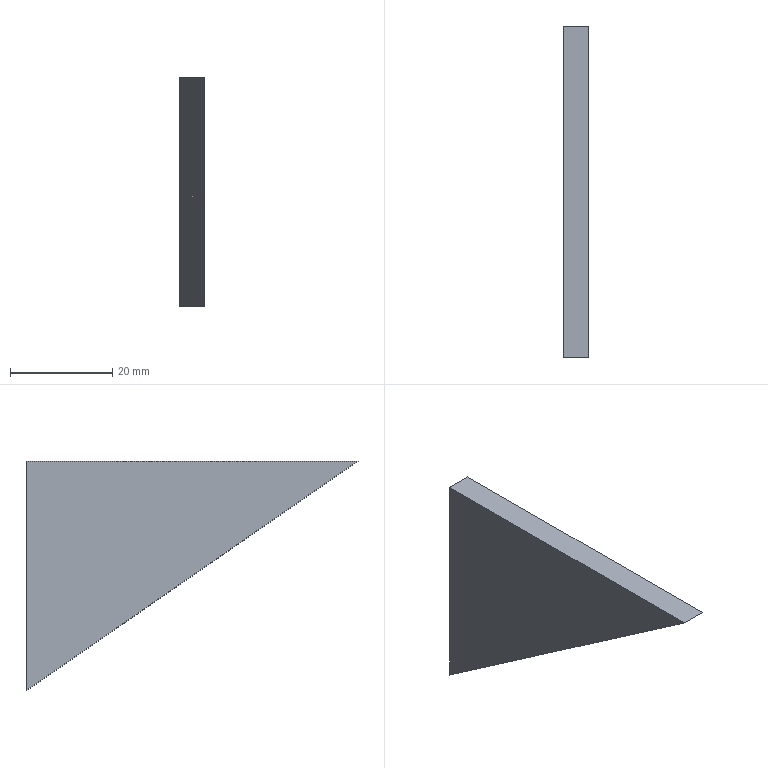Component | NX | FIXED_PLATE_13 | 1 solid | 5 faces | box 5 x 65 x 45 mm | volume 7312 mm3 | plane 5
STEP:
#1=CARTESIAN_POINT('',(0.,0.,0.));
#2=DIRECTION('',(0.,0.,1.));
#3=DIRECTION('',(1.,0.,0.));
#4=AXIS2_PLACEMENT_3D('',#1,#2,#3);
#5=CARTESIAN_POINT('',(1469.254,1356.,781.574));
#6=VERTEX_POINT('',#5);
#7=CARTESIAN_POINT('',(1469.254,1421.,736.574));
#8=VERTEX_POINT('',#7);
#9=CARTESIAN_POINT('',(1469.254,1356.,781.574));
#10=DIRECTION('',(0.,0.8222,-0.5692));
#11=VECTOR('',#10,1.);
#12=LINE('',#9,#11);
#13=CARTESIAN_POINT('',(1464.254,1356.,781.574));
#14=DIRECTION('',(0.,-0.5692,-0.8222));
#15=DIRECTION('',(0.,0.8222,-0.5692));
#16=AXIS2_PLACEMENT_3D('',#13,#14,#15);
#17=PLANE('',#16);
#18=CARTESIAN_POINT('',(0.,5.));
#19=DIRECTION('',(1.,0.));
#20=VECTOR('',#19,1.);
#21=LINE('',#18,#20);
#22=(GEOMETRIC_REPRESENTATION_CONTEXT(2)PARAMETRIC_REPRESENTATION_CONTEXT()REPRESENTATION_CONTEXT('',''));
#23=DEFINITIONAL_REPRESENTATION('',(#21),#22);
#24=PCURVE('',#17,#23);
#25=CARTESIAN_POINT('',(1469.254,0.,0.));
#26=DIRECTION('',(1.,0.,0.));
#27=DIRECTION('',(0.,0.,-1.));
#28=AXIS2_PLACEMENT_3D('',#25,#26,#27);
#29=PLANE('',#28);
#30=CARTESIAN_POINT('',(-781.574,1356.));
#31=DIRECTION('',(0.5692,0.8222));
#32=VECTOR('',#31,1.);
#33=LINE('',#30,#32);
#34=(GEOMETRIC_REPRESENTATION_CONTEXT(2)PARAMETRIC_REPRESENTATION_CONTEXT()REPRESENTATION_CONTEXT('',''));
#35=DEFINITIONAL_REPRESENTATION('',(#33),#34);
#36=PCURVE('',#29,#35);
#37=SURFACE_CURVE('',#12,(#24,#36),.PCURVE_S1.);
#38=EDGE_CURVE('',#6,#8,#37,.T.);
#39=ORIENTED_EDGE('',*,*,#38,.F.);
#40=CARTESIAN_POINT('',(1464.254,1356.,781.574));
#41=VERTEX_POINT('',#40);
#42=CARTESIAN_POINT('',(1464.254,1356.,781.574));
#43=DIRECTION('',(1.,0.,0.));
#44=VECTOR('',#43,1.);
#45=LINE('',#42,#44);
#46=CARTESIAN_POINT('',(0.,0.));
#47=DIRECTION('',(0.,1.));
#48=VECTOR('',#47,1.);
#49=LINE('',#46,#48);
#50=(GEOMETRIC_REPRESENTATION_CONTEXT(2)PARAMETRIC_REPRESENTATION_CONTEXT()REPRESENTATION_CONTEXT('',''));
#51=DEFINITIONAL_REPRESENTATION('',(#49),#50);
#52=PCURVE('',#17,#51);
#53=CARTESIAN_POINT('',(1464.254,1421.,781.574));
#54=DIRECTION('',(0.,0.,1.));
#55=DIRECTION('',(1.,0.,0.));
#56=AXIS2_PLACEMENT_3D('',#53,#54,#55);
#57=PLANE('',#56);
#58=CARTESIAN_POINT('',(0.,-65.));
#59=DIRECTION('',(1.,0.));
#60=VECTOR('',#59,1.);
#61=LINE('',#58,#60);
#62=(GEOMETRIC_REPRESENTATION_CONTEXT(2)PARAMETRIC_REPRESENTATION_CONTEXT()REPRESENTATION_CONTEXT('',''));
#63=DEFINITIONAL_REPRESENTATION('',(#61),#62);
#64=PCURVE('',#57,#63);
#65=SURFACE_CURVE('',#45,(#52,#64),.PCURVE_S1.);
#66=EDGE_CURVE('',#41,#6,#65,.T.);
#67=ORIENTED_EDGE('',*,*,#66,.F.);
#68=CARTESIAN_POINT('',(1464.254,1421.,736.574));
#69=VERTEX_POINT('',#68);
#70=CARTESIAN_POINT('',(1464.254,1356.,781.574));
#71=DIRECTION('',(0.,0.8222,-0.5692));
#72=VECTOR('',#71,1.);
#73=LINE('',#70,#72);
#74=CARTESIAN_POINT('',(0.,0.));
#75=DIRECTION('',(1.,0.));
#76=VECTOR('',#75,1.);
#77=LINE('',#74,#76);
#78=(GEOMETRIC_REPRESENTATION_CONTEXT(2)PARAMETRIC_REPRESENTATION_CONTEXT()REPRESENTATION_CONTEXT('',''));
#79=DEFINITIONAL_REPRESENTATION('',(#77),#78);
#80=PCURVE('',#17,#79);
#81=CARTESIAN_POINT('',(1464.254,0.,0.));
#82=DIRECTION('',(1.,0.,0.));
#83=DIRECTION('',(0.,0.,-1.));
#84=AXIS2_PLACEMENT_3D('',#81,#82,#83);
#85=PLANE('',#84);
#86=CARTESIAN_POINT('',(-781.574,1356.));
#87=DIRECTION('',(0.5692,0.8222));
#88=VECTOR('',#87,1.);
#89=LINE('',#86,#88);
#90=(GEOMETRIC_REPRESENTATION_CONTEXT(2)PARAMETRIC_REPRESENTATION_CONTEXT()REPRESENTATION_CONTEXT('',''));
#91=DEFINITIONAL_REPRESENTATION('',(#89),#90);
#92=PCURVE('',#85,#91);
#93=SURFACE_CURVE('',#73,(#80,#92),.PCURVE_S1.);
#94=EDGE_CURVE('',#41,#69,#93,.T.);
#95=ORIENTED_EDGE('',*,*,#94,.T.);
#96=CARTESIAN_POINT('',(1464.254,1421.,736.574));
#97=DIRECTION('',(1.,0.,0.));
#98=VECTOR('',#97,1.);
#99=LINE('',#96,#98);
#100=CARTESIAN_POINT('',(79.057,0.));
#101=DIRECTION('',(0.,1.));
#102=VECTOR('',#101,1.);
#103=LINE('',#100,#102);
#104=(GEOMETRIC_REPRESENTATION_CONTEXT(2)PARAMETRIC_REPRESENTATION_CONTEXT()REPRESENTATION_CONTEXT('',''));
#105=DEFINITIONAL_REPRESENTATION('',(#103),#104);
#106=PCURVE('',#17,#105);
#107=CARTESIAN_POINT('',(1464.254,1421.,736.574));
#108=DIRECTION('',(0.,1.,0.));
#109=DIRECTION('',(0.,0.,1.));
#110=AXIS2_PLACEMENT_3D('',#107,#108,#109);
#111=PLANE('',#110);
#112=CARTESIAN_POINT('',(0.,0.));
#113=DIRECTION('',(0.,1.));
#114=VECTOR('',#113,1.);
#115=LINE('',#112,#114);
#116=(GEOMETRIC_REPRESENTATION_CONTEXT(2)PARAMETRIC_REPRESENTATION_CONTEXT()REPRESENTATION_CONTEXT('',''));
#117=DEFINITIONAL_REPRESENTATION('',(#115),#116);
#118=PCURVE('',#111,#117);
#119=SURFACE_CURVE('',#99,(#106,#118),.PCURVE_S1.);
#120=EDGE_CURVE('',#69,#8,#119,.T.);
#121=ORIENTED_EDGE('',*,*,#120,.T.);
#122=EDGE_LOOP('',(#39,#67,#95,#121));
#123=FACE_BOUND('',#122,.T.);
#124=ADVANCED_FACE('',(#123),#17,.T.);
#125=CARTESIAN_POINT('',(1469.254,1421.,781.574));
#126=VERTEX_POINT('',#125);
#127=CARTESIAN_POINT('',(1469.254,1421.,736.574));
#128=DIRECTION('',(0.,0.,1.));
#129=VECTOR('',#128,1.);
#130=LINE('',#127,#129);
#131=CARTESIAN_POINT('',(0.,5.));
#132=DIRECTION('',(1.,0.));
#133=VECTOR('',#132,1.);
#134=LINE('',#131,#133);
#135=(GEOMETRIC_REPRESENTATION_CONTEXT(2)PARAMETRIC_REPRESENTATION_CONTEXT()REPRESENTATION_CONTEXT('',''));
#136=DEFINITIONAL_REPRESENTATION('',(#134),#135);
#137=PCURVE('',#111,#136);
#138=CARTESIAN_POINT('',(-736.574,1421.));
#139=DIRECTION('',(-1.,0.));
#140=VECTOR('',#139,1.);
#141=LINE('',#138,#140);
#142=(GEOMETRIC_REPRESENTATION_CONTEXT(2)PARAMETRIC_REPRESENTATION_CONTEXT()REPRESENTATION_CONTEXT('',''));
#143=DEFINITIONAL_REPRESENTATION('',(#141),#142);
#144=PCURVE('',#29,#143);
#145=SURFACE_CURVE('',#130,(#137,#144),.PCURVE_S1.);
#146=EDGE_CURVE('',#8,#126,#145,.T.);
#147=ORIENTED_EDGE('',*,*,#146,.F.);
#148=ORIENTED_EDGE('',*,*,#120,.F.);
#149=CARTESIAN_POINT('',(1464.254,1421.,781.574));
#150=VERTEX_POINT('',#149);
#151=CARTESIAN_POINT('',(1464.254,1421.,736.574));
#152=DIRECTION('',(0.,0.,1.));
#153=VECTOR('',#152,1.);
#154=LINE('',#151,#153);
#155=CARTESIAN_POINT('',(0.,0.));
#156=DIRECTION('',(1.,0.));
#157=VECTOR('',#156,1.);
#158=LINE('',#155,#157);
#159=(GEOMETRIC_REPRESENTATION_CONTEXT(2)PARAMETRIC_REPRESENTATION_CONTEXT()REPRESENTATION_CONTEXT('',''));
#160=DEFINITIONAL_REPRESENTATION('',(#158),#159);
#161=PCURVE('',#111,#160);
#162=CARTESIAN_POINT('',(-736.574,1421.));
#163=DIRECTION('',(-1.,0.));
#164=VECTOR('',#163,1.);
#165=LINE('',#162,#164);
#166=(GEOMETRIC_REPRESENTATION_CONTEXT(2)PARAMETRIC_REPRESENTATION_CONTEXT()REPRESENTATION_CONTEXT('',''));
#167=DEFINITIONAL_REPRESENTATION('',(#165),#166);
#168=PCURVE('',#85,#167);
#169=SURFACE_CURVE('',#154,(#161,#168),.PCURVE_S1.);
#170=EDGE_CURVE('',#69,#150,#169,.T.);
#171=ORIENTED_EDGE('',*,*,#170,.T.);
#172=CARTESIAN_POINT('',(1464.254,1421.,781.574));
#173=DIRECTION('',(1.,0.,0.));
#174=VECTOR('',#173,1.);
#175=LINE('',#172,#174);
#176=CARTESIAN_POINT('',(45.,0.));
#177=DIRECTION('',(0.,1.));
#178=VECTOR('',#177,1.);
#179=LINE('',#176,#178);
#180=(GEOMETRIC_REPRESENTATION_CONTEXT(2)PARAMETRIC_REPRESENTATION_CONTEXT()REPRESENTATION_CONTEXT('',''));
#181=DEFINITIONAL_REPRESENTATION('',(#179),#180);
#182=PCURVE('',#111,#181);
#183=CARTESIAN_POINT('',(0.,0.));
#184=DIRECTION('',(1.,0.));
#185=VECTOR('',#184,1.);
#186=LINE('',#183,#185);
#187=(GEOMETRIC_REPRESENTATION_CONTEXT(2)PARAMETRIC_REPRESENTATION_CONTEXT()REPRESENTATION_CONTEXT('',''));
#188=DEFINITIONAL_REPRESENTATION('',(#186),#187);
#189=PCURVE('',#57,#188);
#190=SURFACE_CURVE('',#175,(#182,#189),.PCURVE_S1.);
#191=EDGE_CURVE('',#150,#126,#190,.T.);
#192=ORIENTED_EDGE('',*,*,#191,.T.);
#193=EDGE_LOOP('',(#147,#148,#171,#192));
#194=FACE_BOUND('',#193,.T.);
#195=ADVANCED_FACE('',(#194),#111,.T.);
#196=CARTESIAN_POINT('',(1469.254,1421.,781.574));
#197=DIRECTION('',(0.,-1.,0.));
#198=VECTOR('',#197,1.);
#199=LINE('',#196,#198);
#200=CARTESIAN_POINT('',(5.,0.));
#201=DIRECTION('',(0.,-1.));
#202=VECTOR('',#201,1.);
#203=LINE('',#200,#202);
#204=(GEOMETRIC_REPRESENTATION_CONTEXT(2)PARAMETRIC_REPRESENTATION_CONTEXT()REPRESENTATION_CONTEXT('',''));
#205=DEFINITIONAL_REPRESENTATION('',(#203),#204);
#206=PCURVE('',#57,#205);
#207=CARTESIAN_POINT('',(-781.574,1421.));
#208=DIRECTION('',(0.,-1.));
#209=VECTOR('',#208,1.);
#210=LINE('',#207,#209);
#211=(GEOMETRIC_REPRESENTATION_CONTEXT(2)PARAMETRIC_REPRESENTATION_CONTEXT()REPRESENTATION_CONTEXT('',''));
#212=DEFINITIONAL_REPRESENTATION('',(#210),#211);
#213=PCURVE('',#29,#212);
#214=SURFACE_CURVE('',#199,(#206,#213),.PCURVE_S1.);
#215=EDGE_CURVE('',#126,#6,#214,.T.);
#216=ORIENTED_EDGE('',*,*,#215,.F.);
#217=ORIENTED_EDGE('',*,*,#191,.F.);
#218=CARTESIAN_POINT('',(1464.254,1421.,781.574));
#219=DIRECTION('',(0.,-1.,0.));
#220=VECTOR('',#219,1.);
#221=LINE('',#218,#220);
#222=CARTESIAN_POINT('',(0.,0.));
#223=DIRECTION('',(0.,-1.));
#224=VECTOR('',#223,1.);
#225=LINE('',#222,#224);
#226=(GEOMETRIC_REPRESENTATION_CONTEXT(2)PARAMETRIC_REPRESENTATION_CONTEXT()REPRESENTATION_CONTEXT('',''));
#227=DEFINITIONAL_REPRESENTATION('',(#225),#226);
#228=PCURVE('',#57,#227);
#229=CARTESIAN_POINT('',(-781.574,1421.));
#230=DIRECTION('',(0.,-1.));
#231=VECTOR('',#230,1.);
#232=LINE('',#229,#231);
#233=(GEOMETRIC_REPRESENTATION_CONTEXT(2)PARAMETRIC_REPRESENTATION_CONTEXT()REPRESENTATION_CONTEXT('',''));
#234=DEFINITIONAL_REPRESENTATION('',(#232),#233);
#235=PCURVE('',#85,#234);
#236=SURFACE_CURVE('',#221,(#228,#235),.PCURVE_S1.);
#237=EDGE_CURVE('',#150,#41,#236,.T.);
#238=ORIENTED_EDGE('',*,*,#237,.T.);
#239=ORIENTED_EDGE('',*,*,#66,.T.);
#240=EDGE_LOOP('',(#216,#217,#238,#239));
#241=FACE_BOUND('',#240,.T.);
#242=ADVANCED_FACE('',(#241),#57,.T.);
#243=ORIENTED_EDGE('',*,*,#94,.F.);
#244=ORIENTED_EDGE('',*,*,#237,.F.);
#245=ORIENTED_EDGE('',*,*,#170,.F.);
#246=EDGE_LOOP('',(#243,#244,#245));
#247=FACE_BOUND('',#246,.T.);
#248=ADVANCED_FACE('',(#247),#85,.F.);
#249=ORIENTED_EDGE('',*,*,#38,.T.);
#250=ORIENTED_EDGE('',*,*,#146,.T.);
#251=ORIENTED_EDGE('',*,*,#215,.T.);
#252=EDGE_LOOP('',(#249,#250,#251));
#253=FACE_BOUND('',#252,.T.);
#254=ADVANCED_FACE('',(#253),#29,.T.);
#255=CLOSED_SHELL('',(#124,#195,#242,#248,#254));
#256=MANIFOLD_SOLID_BREP('',#255);
#257=(LENGTH_UNIT()NAMED_UNIT(*)SI_UNIT(.MILLI.,.METRE.));
#258=UNCERTAINTY_MEASURE_WITH_UNIT(LENGTH_MEASURE(0.0000001),#257,'','');
#259=(NAMED_UNIT(*)PLANE_ANGLE_UNIT()SI_UNIT($,.RADIAN.));
#260=(NAMED_UNIT(*)SI_UNIT($,.STERADIAN.)SOLID_ANGLE_UNIT());
#261=(GEOMETRIC_REPRESENTATION_CONTEXT(3)GLOBAL_UNCERTAINTY_ASSIGNED_CONTEXT((#258))GLOBAL_UNIT_ASSIGNED_CONTEXT((#257,#259,#260))REPRESENTATION_CONTEXT('',''));
#262=ADVANCED_BREP_SHAPE_REPRESENTATION('',(#4,#256),#261);